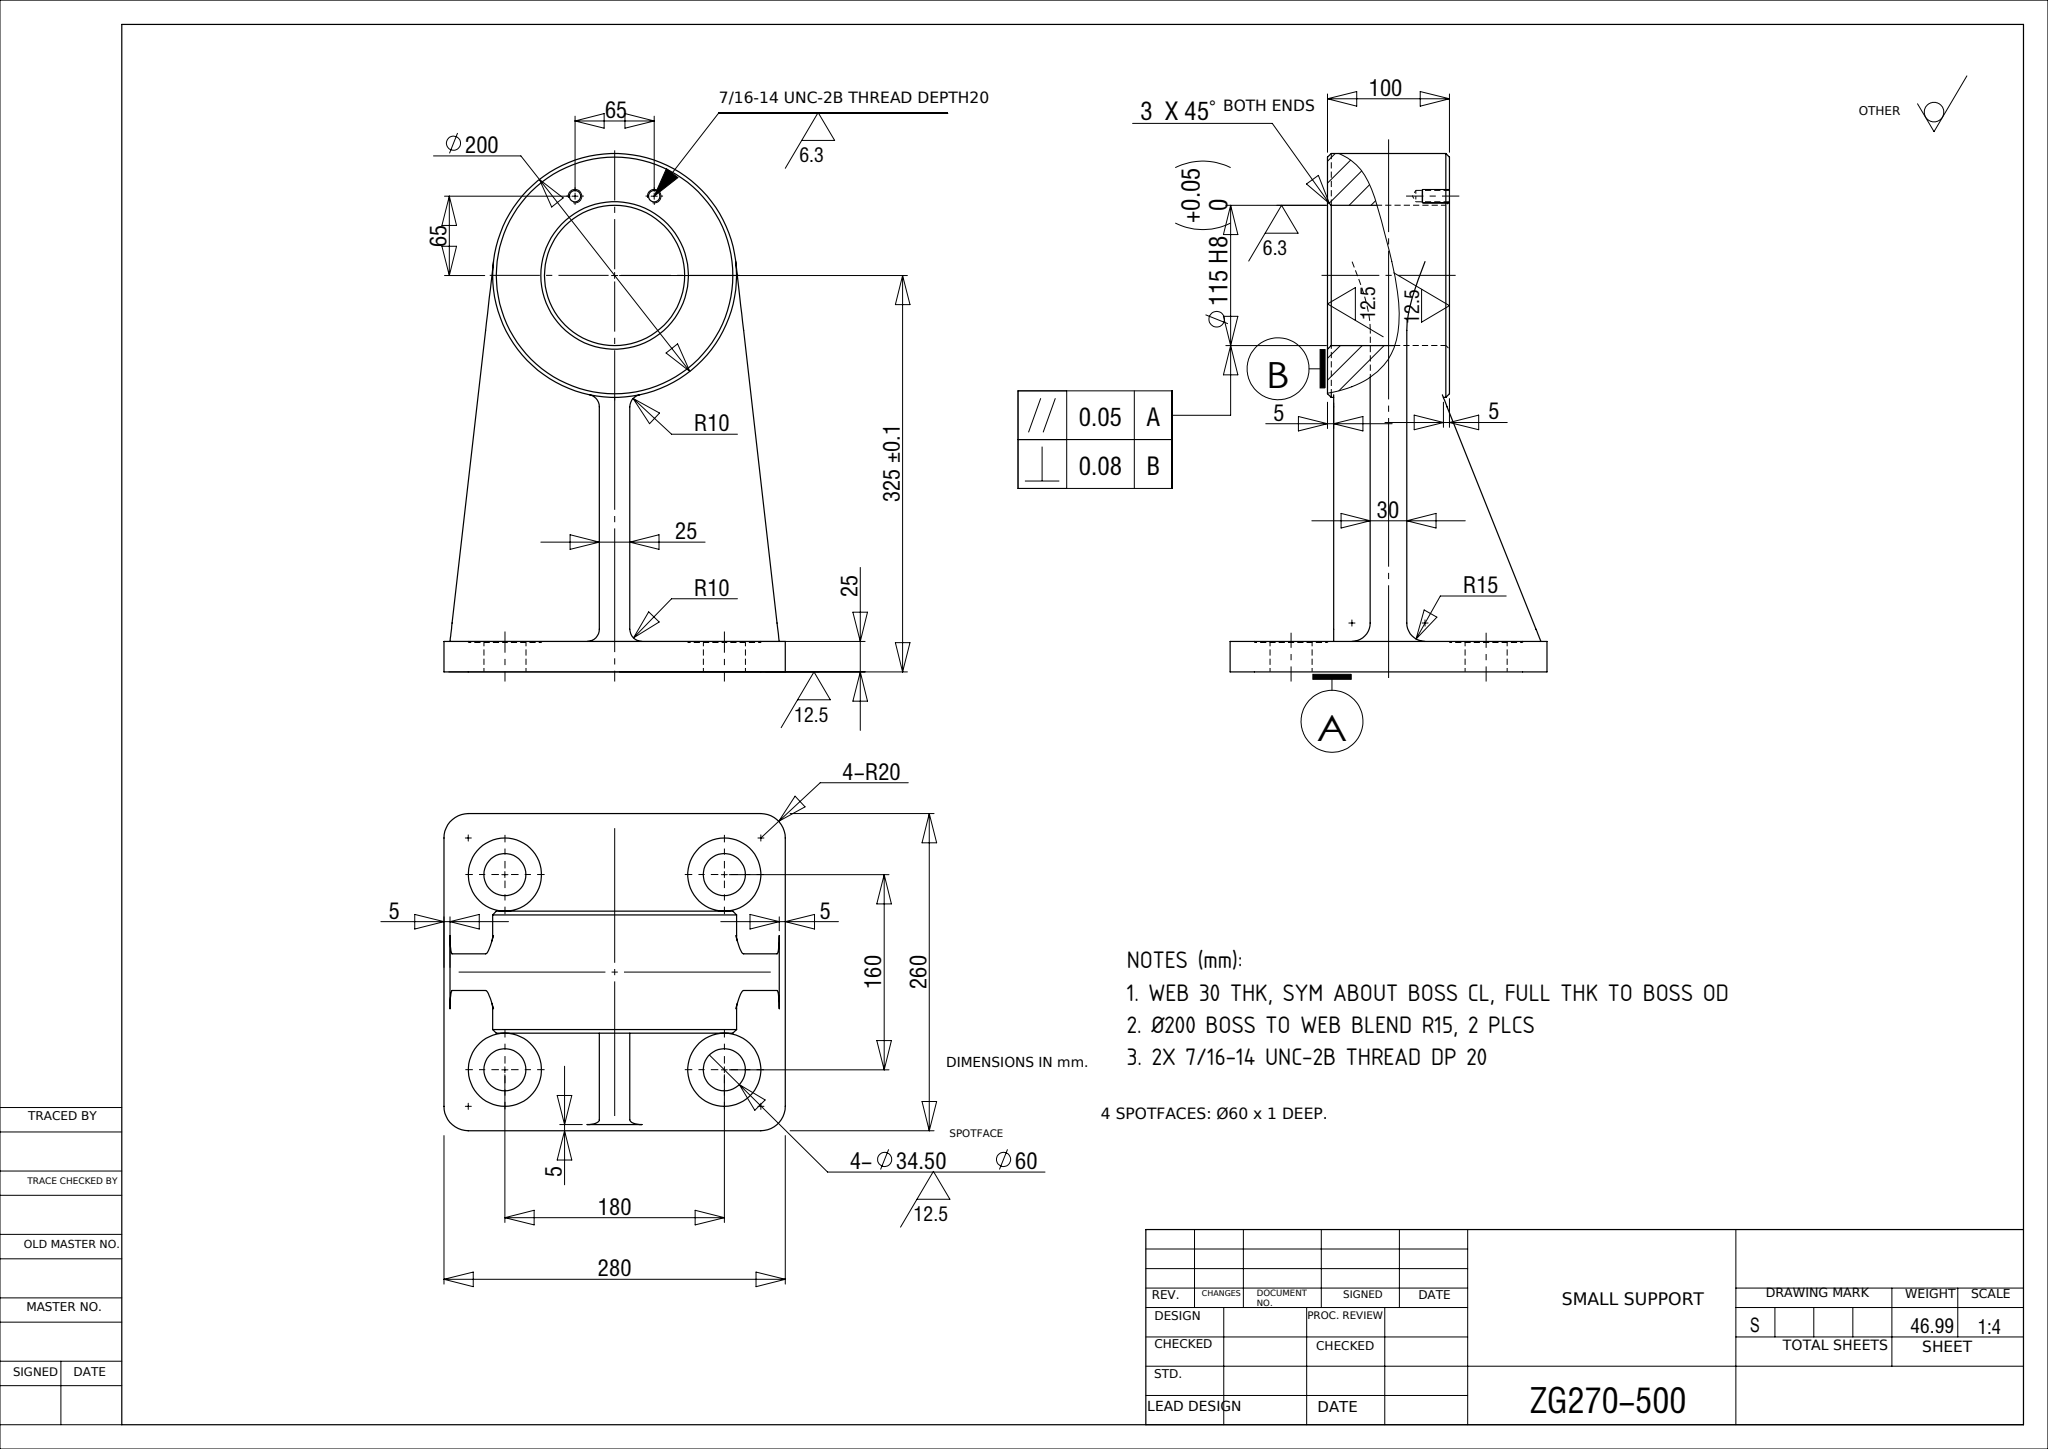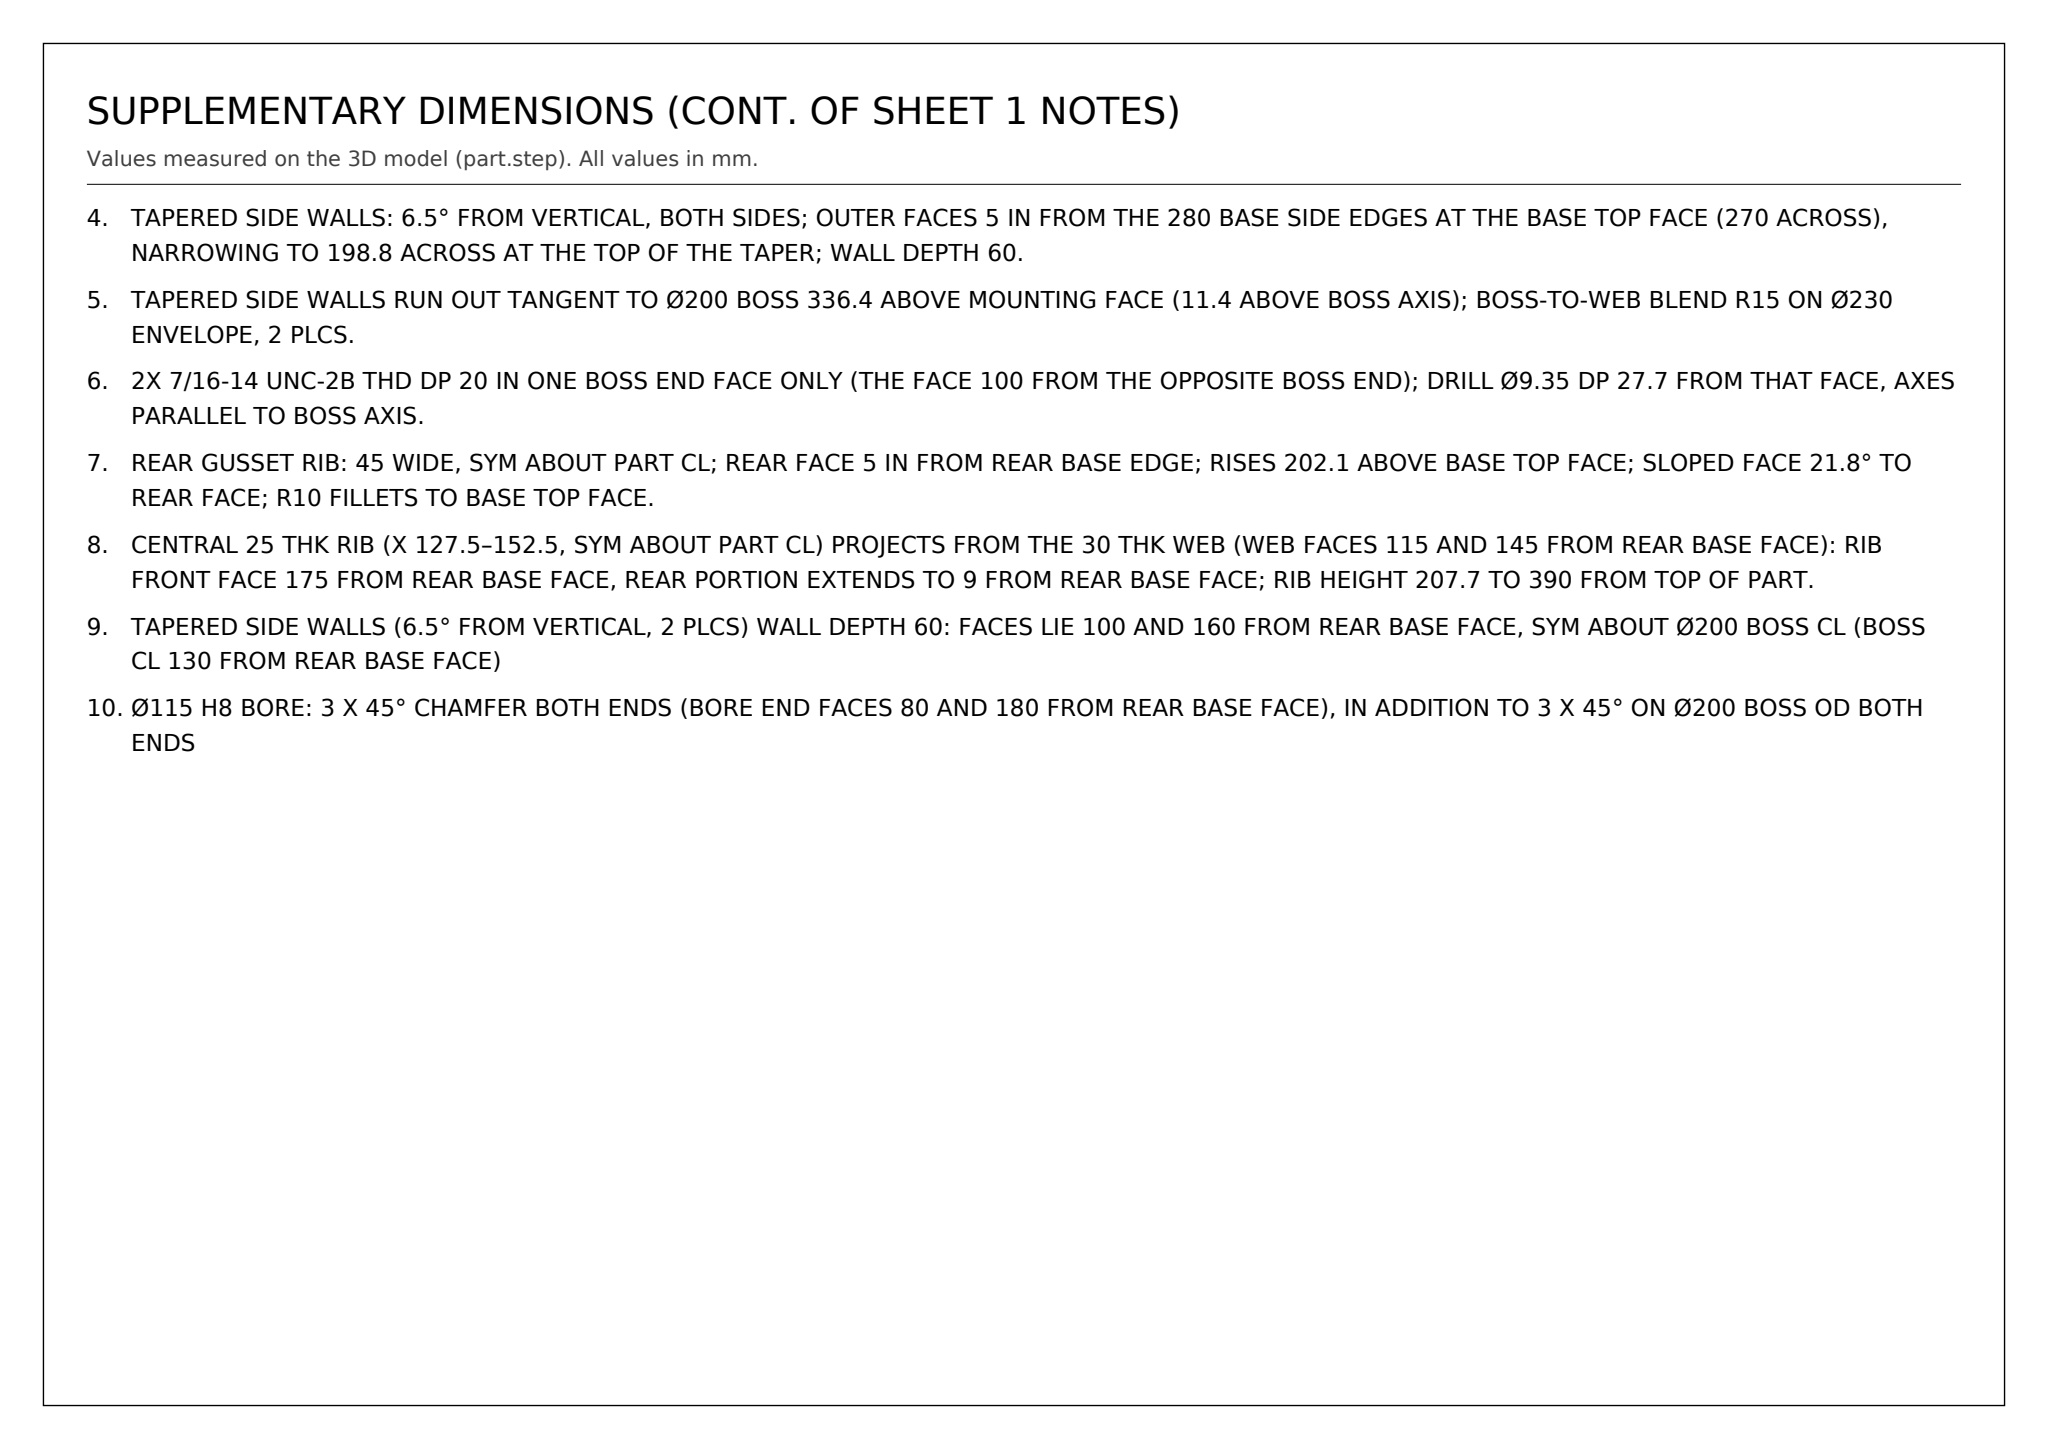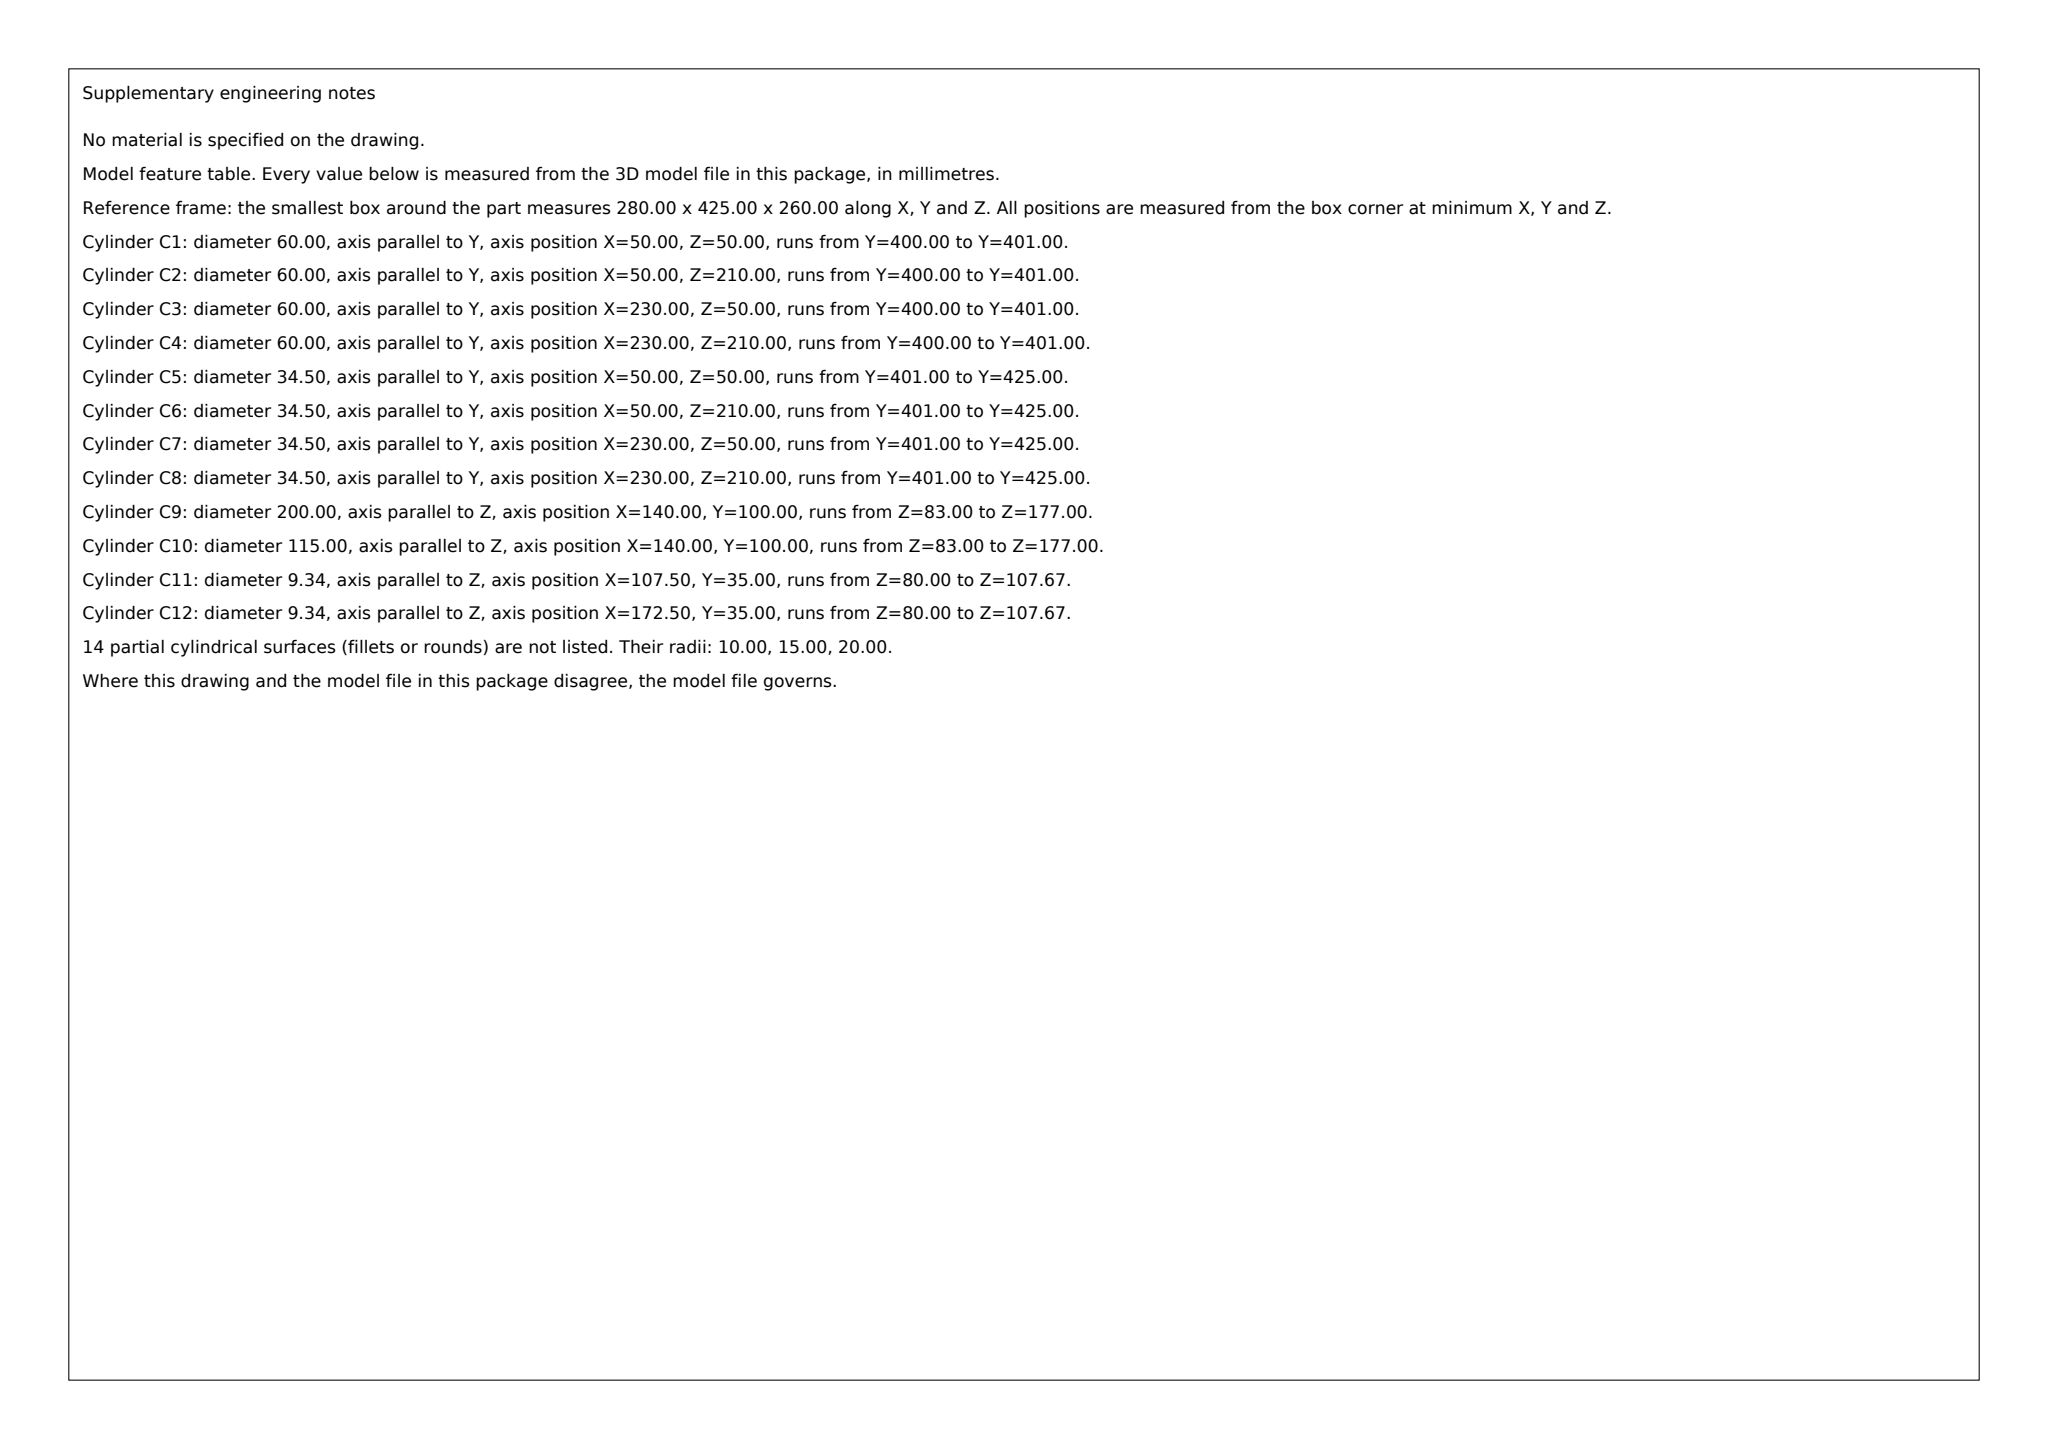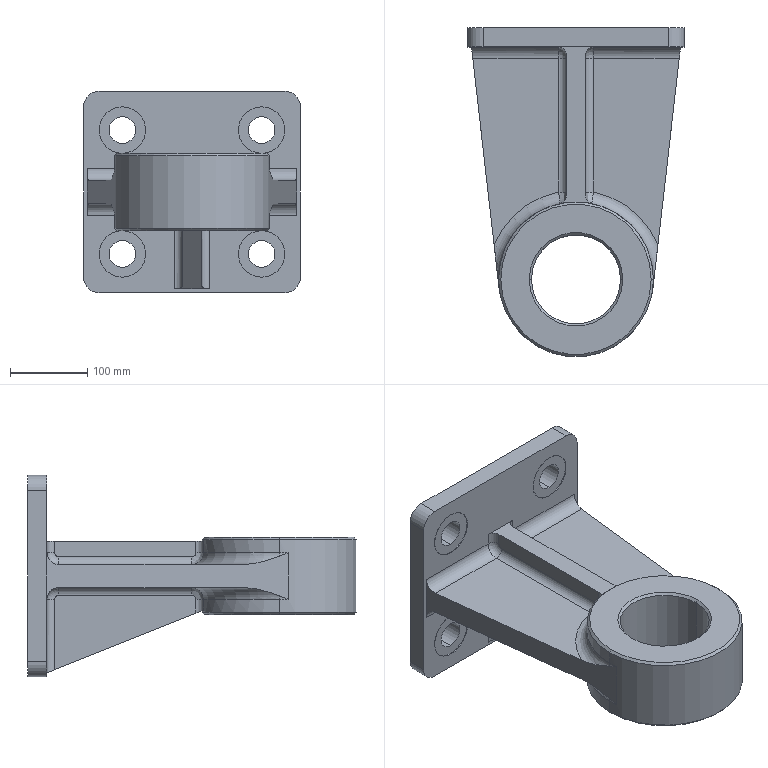Part | SolidWorks | mm | material ZG270-500 | 1 solid | 95 faces | box 280 x 425 x 260 mm | volume 6024074 mm3 | cylinder 45 | plane 24 | cone 12 | torus 10 | spline 4 | commonest cylinder face diameters 20 x12 60 x8 34.5 x8 9.347 x4 30 x4 40 x4 200 x3 115 x2
Drawing notes:
WEB 30 THK, SYM ABOUT BOSS CL, FULL THK TO BOSS OD | from the solid: axis_planes z=115 (x2) and z=145 (x2) -> 30 thk; boss axis z=130 so web centered; boss faces z=80/180 (100 wide)
Ø200 BOSS TO WEB BLEND R15, 2 PLCS | from the solid: fillet_radii [15.0,6]: 4 at web-to-base (Ø30 fillet cyls y=385, z=100/160); remaining 2 are boss-to-web blends
2X 7/16-14 UNC-2B THREAD DP 20 | from the solid: cylinders Ø9.347 axis z at (107.5,35) and (172.5,35), L=27.67, with 118° drill point cones (4 faces = 2 holes)
TAPERED SIDE WALLS: 6.5° FROM VERTICAL, BOTH SIDES; OUTER FACES 5 IN FROM THE 280 BASE SIDE EDGES AT THE BASE TOP FACE (270 ACROSS), NARROWING TO 198.8 ACROSS AT THE TOP OF THE TAPER; WALL DEPTH 60. | from the solid: inclined_planes angle_to_xyz_axes [6.5,83.5,90], bbox_from [5.0,88.6,100.0] and [239.4,88.6,100.0], size [35.6,311.4,60.0]
TAPERED SIDE WALLS RUN OUT TANGENT TO Ø200 BOSS 336.4 ABOVE MOUNTING FACE (11.4 ABOVE BOSS AXIS); BOSS-TO-WEB BLEND R15 ON Ø230 ENVELOPE, 2 PLCS. | from the solid: inclined plane y-extent 88.6–400 with base mounting face at y=425; tori [minor_r 15, major 115]
2X 7/16-14 UNC-2B THD DP 20 IN ONE BOSS END FACE ONLY (THE FACE 100 FROM THE OPPOSITE BOSS END); DRILL Ø9.35 DP 27.7 FROM THAT FACE, AXES PARALLEL TO BOSS AXIS. | from the solid: cylinders hole/bore Ø9.35 axis z at (107.5,35) and (172.5,35), from 80.0 to 107.7; boss outer Ø200 spans z 80–180
REAR GUSSET RIB: 45 WIDE, SYM ABOUT PART CL; REAR FACE 5 IN FROM REAR BASE EDGE; RISES 202.1 ABOVE BASE TOP FACE; SLOPED FACE 21.8° TO REAR FACE; R10 FILLETS TO BASE TOP FACE. | from the solid: inclined_planes angle [90,68.2,21.8], bbox_from [117.5,197.9,5.0], size [45,202.1,80.8]; concave Ø20 arcs axis z at x=117.5/162.5, y=390, from 5.0 to 100.0
CENTRAL 25 THK RIB (X 127.5–152.5, SYM ABOUT PART CL) PROJECTS FROM THE 30 THK WEB (WEB FACES 115 AND 145 FROM REAR BASE FACE): RIB FRONT FACE 175 FROM REAR BASE FACE, REAR PORTION EXTENDS TO 9 FROM REAR BASE FACE; RIB HEIGHT 207.7 TO 390 FROM TOP OF PART. | from the solid: axis_planes x=127.5 and x=152.5, extents z 155–175 and z 9–105, y 207.7–390; axis_planes z=115 and z=145 (web faces); plane z=175 x 117.5–162.5
TAPERED SIDE WALLS (6.5° FROM VERTICAL, 2 PLCS) WALL DEPTH 60: FACES LIE 100 AND 160 FROM REAR BASE FACE, SYM ABOUT Ø200 BOSS CL (BOSS CL 130 FROM REAR BASE FACE) | from the solid: inclined_planes 6.5°/83.5°/90°, bbox_from z=100, size z=60 (2 plcs); Ø115 bore axis z from 83 to 177 (CL z=130)
Ø115 H8 BORE: 3 X 45° CHAMFER BOTH ENDS (BORE END FACES 80 AND 180 FROM REAR BASE FACE), IN ADDITION TO 3 X 45° ON Ø200 BOSS OD BOTH ENDS | from the solid: cones 90° included, ref dia 115 at z=177 size 3 and ref dia 121 at z=80 size 3 (bore ends); cones 90° ref dia 194/200 at z=177/80 (boss OD)